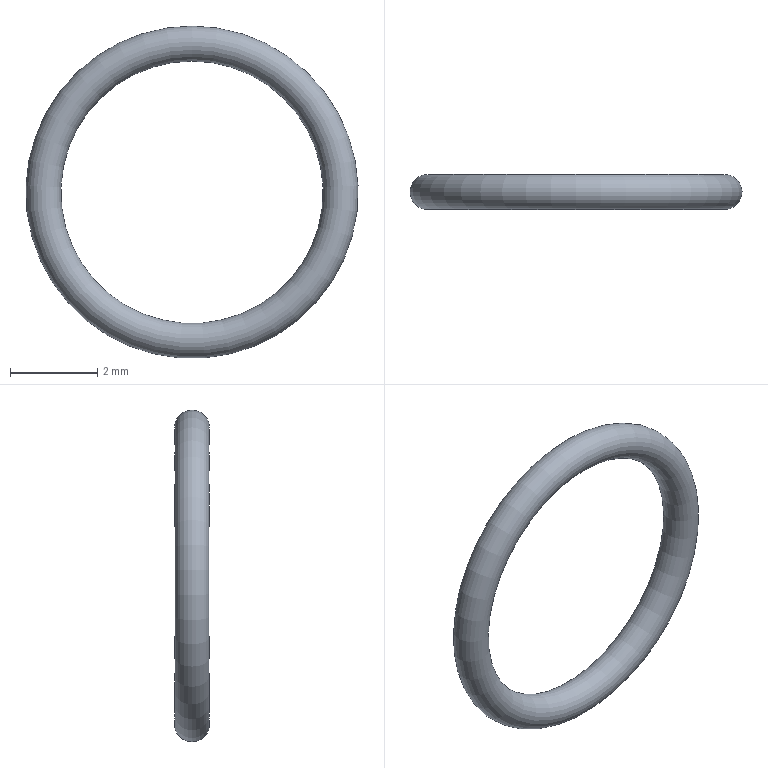Component | NX | O_RING | 1 solid | 1 faces | box 7.6 x 0.8 x 7.6 mm | volume 11 mm3 | torus 1
STEP:
#1=CARTESIAN_POINT('',(0.,0.,0.));
#2=DIRECTION('',(0.,0.,1.));
#3=DIRECTION('',(1.,0.,0.));
#4=AXIS2_PLACEMENT_3D('',#1,#2,#3);
#5=CARTESIAN_POINT('',(13.994,-104.182,3.8));
#6=VERTEX_POINT('',#5);
#7=CARTESIAN_POINT('',(13.994,-104.182,3.4));
#8=DIRECTION('',(-1.,0.,0.));
#9=DIRECTION('',(0.,0.,1.));
#10=AXIS2_PLACEMENT_3D('',#7,#8,#9);
#11=CIRCLE('',#10,0.4);
#12=CARTESIAN_POINT('',(13.994,-104.182,-0.));
#13=DIRECTION('',(0.,1.,0.));
#14=DIRECTION('',(0.,0.,1.));
#15=AXIS2_PLACEMENT_3D('',#12,#13,#14);
#16=TOROIDAL_SURFACE('',#15,3.4,0.4);
#17=CARTESIAN_POINT('',(0.,0.));
#18=DIRECTION('',(0.,1.));
#19=VECTOR('',#18,1.);
#20=LINE('',#17,#19);
#21=(GEOMETRIC_REPRESENTATION_CONTEXT(2)PARAMETRIC_REPRESENTATION_CONTEXT()REPRESENTATION_CONTEXT('',''));
#22=DEFINITIONAL_REPRESENTATION('',(#20),#21);
#23=PCURVE('',#16,#22);
#24=CARTESIAN_POINT('',(6.283,0.));
#25=DIRECTION('',(0.,1.));
#26=VECTOR('',#25,1.);
#27=LINE('',#24,#26);
#28=(GEOMETRIC_REPRESENTATION_CONTEXT(2)PARAMETRIC_REPRESENTATION_CONTEXT()REPRESENTATION_CONTEXT('',''));
#29=DEFINITIONAL_REPRESENTATION('',(#27),#28);
#30=PCURVE('',#16,#29);
#31=SEAM_CURVE('',#11,(#23,#30),.PCURVE_S1.);
#32=EDGE_CURVE('',#6,#6,#31,.T.);
#33=ORIENTED_EDGE('',*,*,#32,.F.);
#34=CARTESIAN_POINT('',(13.994,-104.182,-0.));
#35=DIRECTION('',(0.,1.,0.));
#36=DIRECTION('',(0.,0.,1.));
#37=AXIS2_PLACEMENT_3D('',#34,#35,#36);
#38=CIRCLE('',#37,3.8);
#39=CARTESIAN_POINT('',(0.,0.));
#40=DIRECTION('',(1.,0.));
#41=VECTOR('',#40,1.);
#42=LINE('',#39,#41);
#43=(GEOMETRIC_REPRESENTATION_CONTEXT(2)PARAMETRIC_REPRESENTATION_CONTEXT()REPRESENTATION_CONTEXT('',''));
#44=DEFINITIONAL_REPRESENTATION('',(#42),#43);
#45=PCURVE('',#16,#44);
#46=CARTESIAN_POINT('',(0.,6.283));
#47=DIRECTION('',(1.,0.));
#48=VECTOR('',#47,1.);
#49=LINE('',#46,#48);
#50=(GEOMETRIC_REPRESENTATION_CONTEXT(2)PARAMETRIC_REPRESENTATION_CONTEXT()REPRESENTATION_CONTEXT('',''));
#51=DEFINITIONAL_REPRESENTATION('',(#49),#50);
#52=PCURVE('',#16,#51);
#53=SEAM_CURVE('',#38,(#45,#52),.PCURVE_S1.);
#54=EDGE_CURVE('',#6,#6,#53,.T.);
#55=ORIENTED_EDGE('',*,*,#54,.T.);
#56=ORIENTED_EDGE('',*,*,#32,.T.);
#57=ORIENTED_EDGE('',*,*,#54,.F.);
#58=EDGE_LOOP('',(#33,#55,#56,#57));
#59=FACE_BOUND('',#58,.T.);
#60=ADVANCED_FACE('',(#59),#16,.T.);
#61=CLOSED_SHELL('',(#60));
#62=MANIFOLD_SOLID_BREP('',#61);
#63=(LENGTH_UNIT()NAMED_UNIT(*)SI_UNIT(.MILLI.,.METRE.));
#64=UNCERTAINTY_MEASURE_WITH_UNIT(LENGTH_MEASURE(0.0000001),#63,'','');
#65=(NAMED_UNIT(*)PLANE_ANGLE_UNIT()SI_UNIT($,.RADIAN.));
#66=(NAMED_UNIT(*)SI_UNIT($,.STERADIAN.)SOLID_ANGLE_UNIT());
#67=(GEOMETRIC_REPRESENTATION_CONTEXT(3)GLOBAL_UNCERTAINTY_ASSIGNED_CONTEXT((#64))GLOBAL_UNIT_ASSIGNED_CONTEXT((#63,#65,#66))REPRESENTATION_CONTEXT('',''));
#68=ADVANCED_BREP_SHAPE_REPRESENTATION('',(#4,#62),#67);